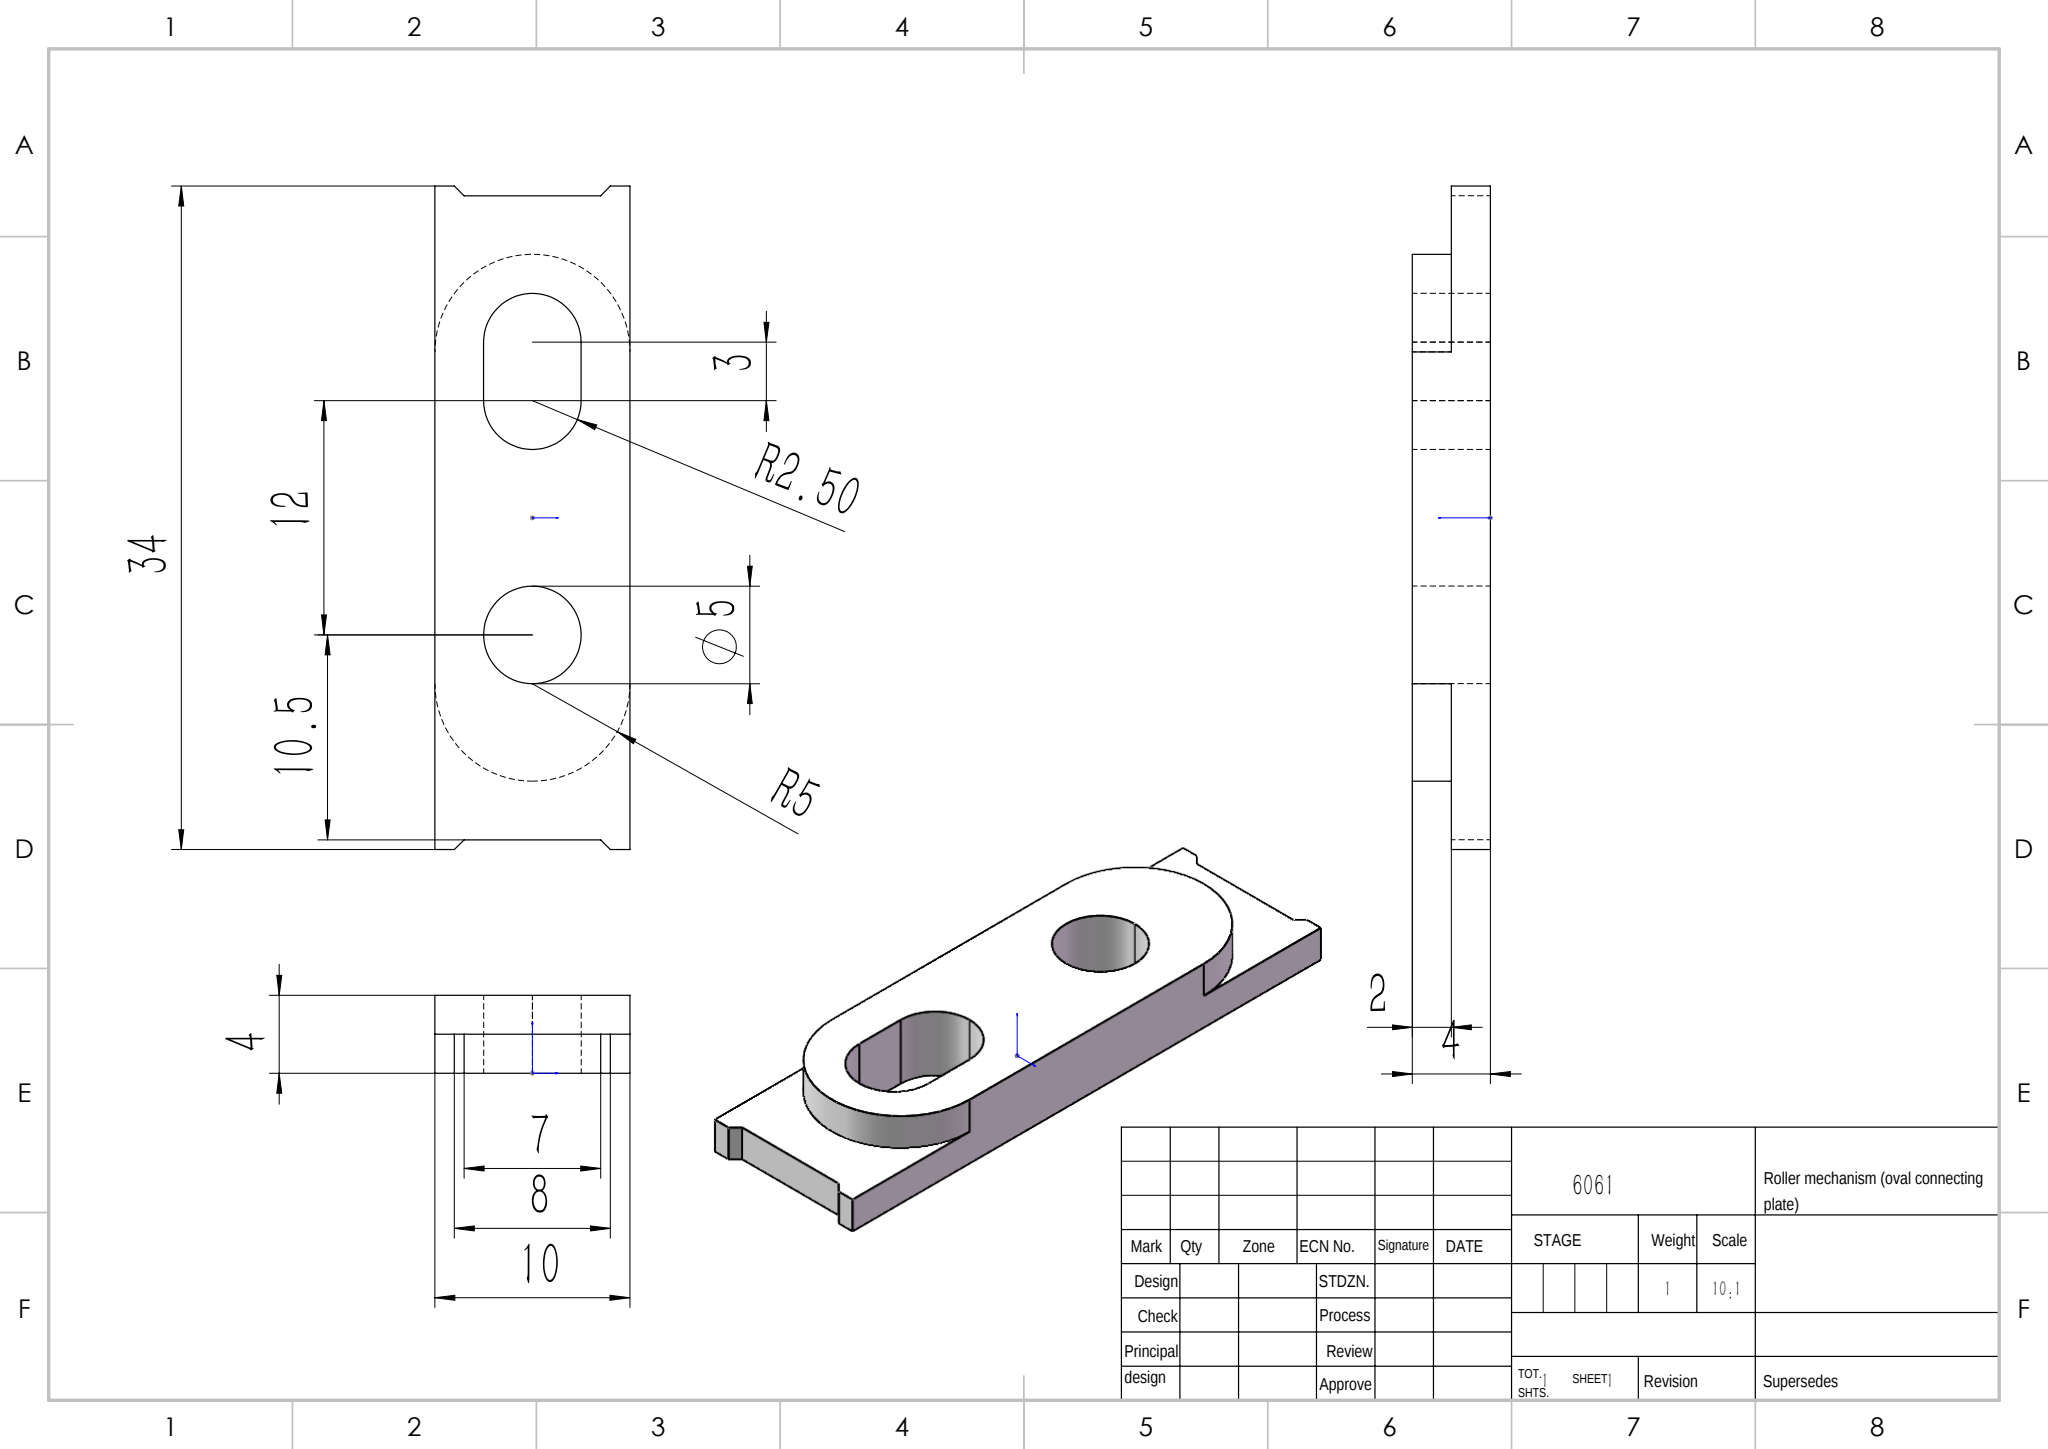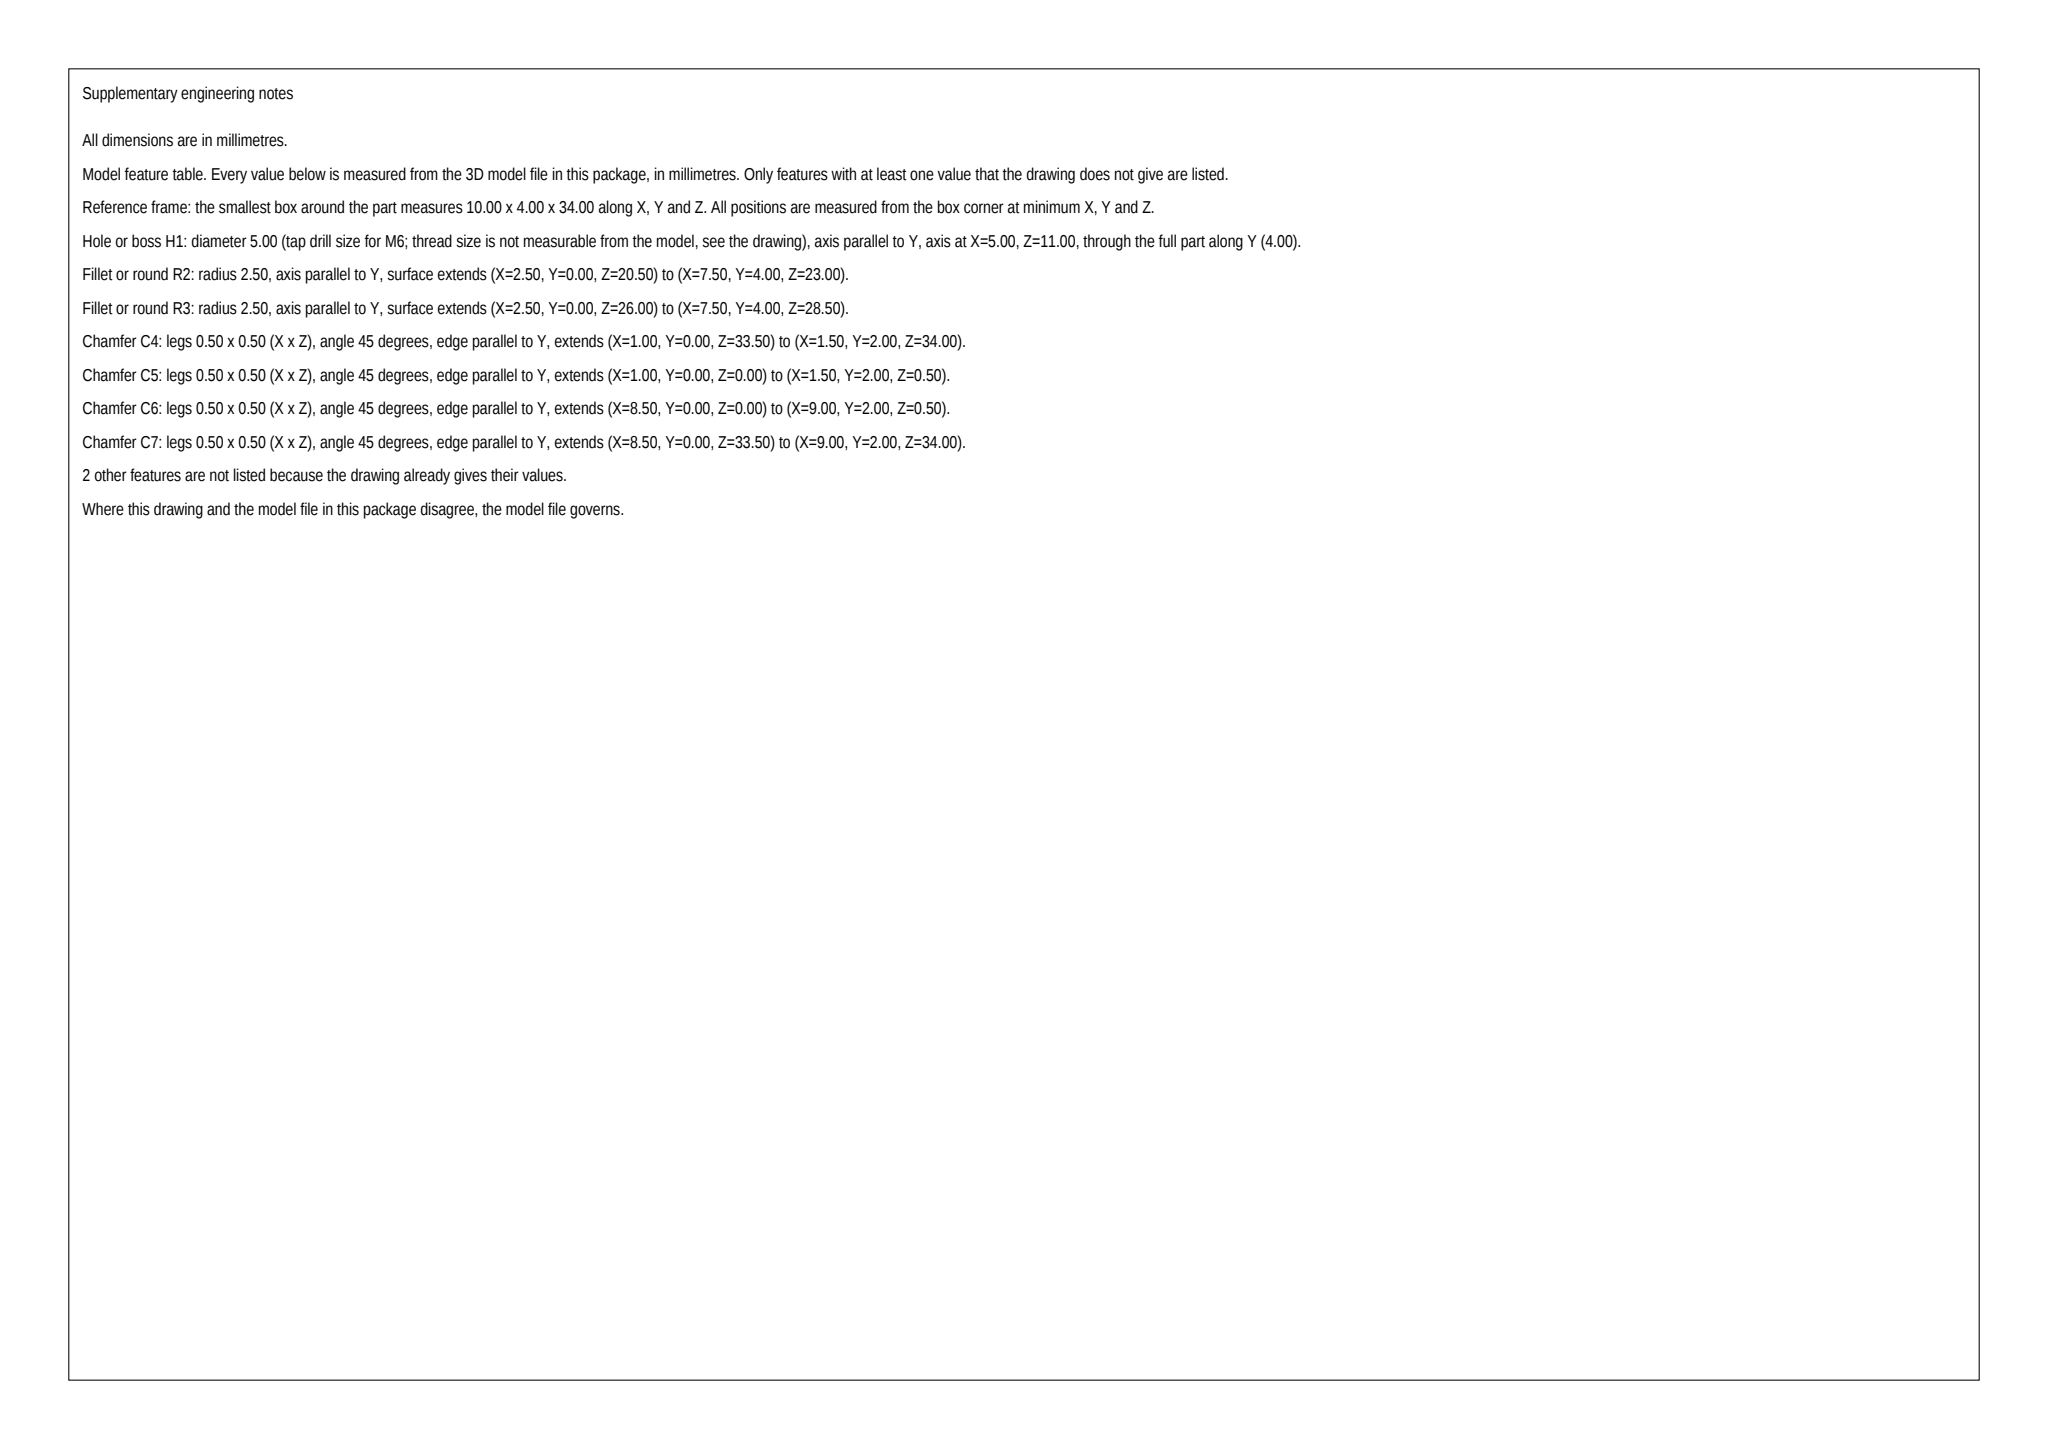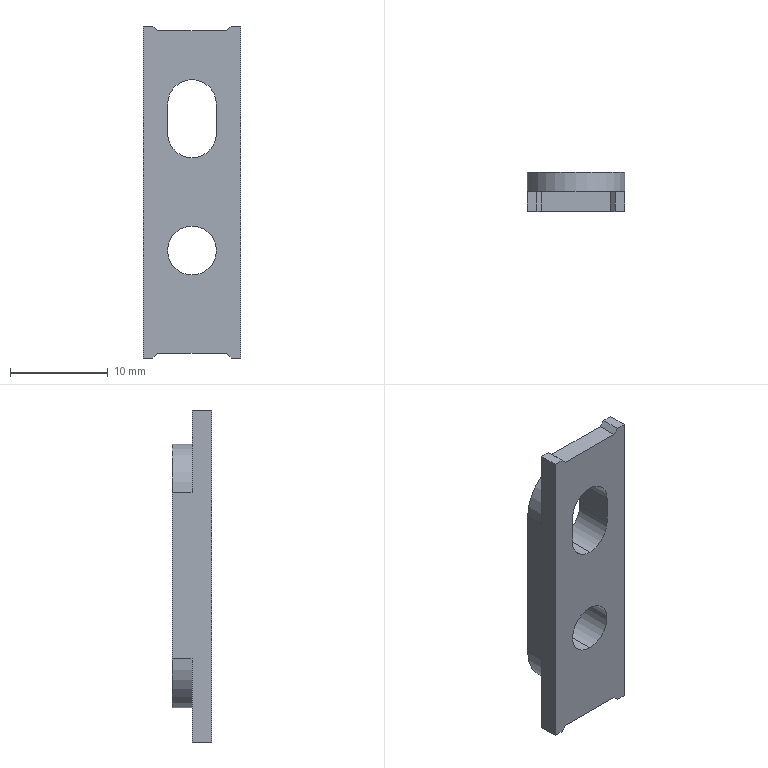Part | SolidWorks | mm | material 6061 | 1 solid | 26 faces | box 10 x 4 x 34 mm | volume 945 mm3 | plane 18 | cylinder 8 | commonest cylinder face diameters 5 x5 10 x3
STEP:
#1=CARTESIAN_POINT('',(2.5,4.,6.));
#2=VERTEX_POINT('',#1);
#3=CARTESIAN_POINT('',(2.5,0.,6.));
#4=VERTEX_POINT('',#3);
#5=CARTESIAN_POINT('',(2.5,4.,6.));
#6=DIRECTION('',(0.,-1.,0.));
#7=VECTOR('',#6,1000.);
#8=LINE('',#5,#7);
#9=EDGE_CURVE('',#2,#4,#8,.T.);
#10=ORIENTED_EDGE('',*,*,#9,.T.);
#11=CARTESIAN_POINT('',(2.5,0.,9.));
#12=VERTEX_POINT('',#11);
#13=CARTESIAN_POINT('',(2.5,0.,-0.));
#14=DIRECTION('',(0.,0.,1.));
#15=VECTOR('',#14,1000.);
#16=LINE('',#13,#15);
#17=EDGE_CURVE('',#4,#12,#16,.T.);
#18=ORIENTED_EDGE('',*,*,#17,.T.);
#19=CARTESIAN_POINT('',(2.5,4.,9.));
#20=VERTEX_POINT('',#19);
#21=CARTESIAN_POINT('',(2.5,4.,9.));
#22=DIRECTION('',(0.,-1.,0.));
#23=VECTOR('',#22,1000.);
#24=LINE('',#21,#23);
#25=EDGE_CURVE('',#20,#12,#24,.T.);
#26=ORIENTED_EDGE('',*,*,#25,.F.);
#27=CARTESIAN_POINT('',(2.5,4.,6.));
#28=DIRECTION('',(-0.,0.,-1.));
#29=VECTOR('',#28,1000.);
#30=LINE('',#27,#29);
#31=EDGE_CURVE('',#20,#2,#30,.T.);
#32=ORIENTED_EDGE('',*,*,#31,.T.);
#33=EDGE_LOOP('',(#10,#18,#26,#32));
#34=FACE_OUTER_BOUND('',#33,.T.);
#35=CARTESIAN_POINT('',(2.5,4.,6.));
#36=DIRECTION('',(-1.,0.,0.));
#37=DIRECTION('',(0.,1.,0.));
#38=AXIS2_PLACEMENT_3D('',#35,#36,#37);
#39=PLANE('',#38);
#40=ADVANCED_FACE('',(#34),#39,.T.);
#41=ORIENTED_EDGE('',*,*,#25,.T.);
#42=CARTESIAN_POINT('',(-2.5,0.,9.));
#43=VERTEX_POINT('',#42);
#44=CARTESIAN_POINT('',(0.,0.,9.));
#45=DIRECTION('',(0.,1.,0.));
#46=DIRECTION('',(0.,0.,1.));
#47=AXIS2_PLACEMENT_3D('',#44,#45,#46);
#48=CIRCLE('',#47,2.5);
#49=EDGE_CURVE('',#43,#12,#48,.T.);
#50=ORIENTED_EDGE('',*,*,#49,.F.);
#51=CARTESIAN_POINT('',(-2.5,4.,9.));
#52=VERTEX_POINT('',#51);
#53=CARTESIAN_POINT('',(-2.5,4.,9.));
#54=DIRECTION('',(0.,-1.,0.));
#55=VECTOR('',#54,1000.);
#56=LINE('',#53,#55);
#57=EDGE_CURVE('',#52,#43,#56,.T.);
#58=ORIENTED_EDGE('',*,*,#57,.F.);
#59=CARTESIAN_POINT('',(0.,4.,9.));
#60=DIRECTION('',(0.,1.,0.));
#61=DIRECTION('',(0.,0.,1.));
#62=AXIS2_PLACEMENT_3D('',#59,#60,#61);
#63=CIRCLE('',#62,2.5);
#64=EDGE_CURVE('',#52,#20,#63,.T.);
#65=ORIENTED_EDGE('',*,*,#64,.T.);
#66=EDGE_LOOP('',(#41,#50,#58,#65));
#67=FACE_OUTER_BOUND('',#66,.T.);
#68=CARTESIAN_POINT('',(0.,4.,9.));
#69=DIRECTION('',(0.,-1.,0.));
#70=DIRECTION('',(0.,0.,-1.));
#71=AXIS2_PLACEMENT_3D('',#68,#69,#70);
#72=CYLINDRICAL_SURFACE('',#71,2.5);
#73=ADVANCED_FACE('',(#67),#72,.F.);
#74=ORIENTED_EDGE('',*,*,#57,.T.);
#75=CARTESIAN_POINT('',(-2.5,0.,6.));
#76=VERTEX_POINT('',#75);
#77=CARTESIAN_POINT('',(-2.5,0.,0.));
#78=DIRECTION('',(0.,0.,1.));
#79=VECTOR('',#78,1000.);
#80=LINE('',#77,#79);
#81=EDGE_CURVE('',#76,#43,#80,.T.);
#82=ORIENTED_EDGE('',*,*,#81,.F.);
#83=CARTESIAN_POINT('',(-2.5,4.,6.));
#84=VERTEX_POINT('',#83);
#85=CARTESIAN_POINT('',(-2.5,4.,6.));
#86=DIRECTION('',(0.,-1.,0.));
#87=VECTOR('',#86,1000.);
#88=LINE('',#85,#87);
#89=EDGE_CURVE('',#84,#76,#88,.T.);
#90=ORIENTED_EDGE('',*,*,#89,.F.);
#91=CARTESIAN_POINT('',(-2.5,4.,6.));
#92=DIRECTION('',(0.,0.,1.));
#93=VECTOR('',#92,1000.);
#94=LINE('',#91,#93);
#95=EDGE_CURVE('',#84,#52,#94,.T.);
#96=ORIENTED_EDGE('',*,*,#95,.T.);
#97=EDGE_LOOP('',(#74,#82,#90,#96));
#98=FACE_OUTER_BOUND('',#97,.T.);
#99=CARTESIAN_POINT('',(-2.5,4.,6.));
#100=DIRECTION('',(1.,0.,-0.));
#101=DIRECTION('',(-0.,0.,-1.));
#102=AXIS2_PLACEMENT_3D('',#99,#100,#101);
#103=PLANE('',#102);
#104=ADVANCED_FACE('',(#98),#103,.T.);
#105=CARTESIAN_POINT('',(0.,4.,3.5));
#106=VERTEX_POINT('',#105);
#107=CARTESIAN_POINT('',(0.,0.,3.5));
#108=VERTEX_POINT('',#107);
#109=CARTESIAN_POINT('',(0.,4.,3.5));
#110=DIRECTION('',(0.,-1.,0.));
#111=VECTOR('',#110,1000.);
#112=LINE('',#109,#111);
#113=EDGE_CURVE('',#106,#108,#112,.T.);
#114=ORIENTED_EDGE('',*,*,#113,.F.);
#115=CARTESIAN_POINT('',(0.,4.,6.));
#116=DIRECTION('',(0.,1.,0.));
#117=DIRECTION('',(0.,0.,1.));
#118=AXIS2_PLACEMENT_3D('',#115,#116,#117);
#119=CIRCLE('',#118,2.5);
#120=EDGE_CURVE('',#106,#84,#119,.T.);
#121=ORIENTED_EDGE('',*,*,#120,.T.);
#122=ORIENTED_EDGE('',*,*,#89,.T.);
#123=CARTESIAN_POINT('',(0.,0.,6.));
#124=DIRECTION('',(0.,1.,0.));
#125=DIRECTION('',(0.,0.,1.));
#126=AXIS2_PLACEMENT_3D('',#123,#124,#125);
#127=CIRCLE('',#126,2.5);
#128=EDGE_CURVE('',#108,#76,#127,.T.);
#129=ORIENTED_EDGE('',*,*,#128,.F.);
#130=EDGE_LOOP('',(#114,#121,#122,#129));
#131=FACE_OUTER_BOUND('',#130,.T.);
#132=CARTESIAN_POINT('',(0.,4.,6.));
#133=DIRECTION('',(0.,-1.,0.));
#134=DIRECTION('',(0.,0.,-1.));
#135=AXIS2_PLACEMENT_3D('',#132,#133,#134);
#136=CYLINDRICAL_SURFACE('',#135,2.5);
#137=ADVANCED_FACE('',(#131),#136,.F.);
#138=CARTESIAN_POINT('',(0.,4.,-3.5));
#139=VERTEX_POINT('',#138);
#140=CARTESIAN_POINT('',(0.,0.,-3.5));
#141=VERTEX_POINT('',#140);
#142=CARTESIAN_POINT('',(0.,4.,-3.5));
#143=DIRECTION('',(0.,-1.,0.));
#144=VECTOR('',#143,1000.);
#145=LINE('',#142,#144);
#146=EDGE_CURVE('',#139,#141,#145,.T.);
#147=ORIENTED_EDGE('',*,*,#146,.F.);
#148=CARTESIAN_POINT('',(0.,4.,-8.5));
#149=VERTEX_POINT('',#148);
#150=CARTESIAN_POINT('',(0.,4.,-6.));
#151=DIRECTION('',(0.,1.,0.));
#152=DIRECTION('',(0.,0.,1.));
#153=AXIS2_PLACEMENT_3D('',#150,#151,#152);
#154=CIRCLE('',#153,2.5);
#155=EDGE_CURVE('',#139,#149,#154,.T.);
#156=ORIENTED_EDGE('',*,*,#155,.T.);
#157=CARTESIAN_POINT('',(0.,0.,-8.5));
#158=VERTEX_POINT('',#157);
#159=CARTESIAN_POINT('',(0.,4.,-8.5));
#160=DIRECTION('',(0.,-1.,0.));
#161=VECTOR('',#160,1000.);
#162=LINE('',#159,#161);
#163=EDGE_CURVE('',#149,#158,#162,.T.);
#164=ORIENTED_EDGE('',*,*,#163,.T.);
#165=CARTESIAN_POINT('',(0.,0.,-6.));
#166=DIRECTION('',(0.,1.,0.));
#167=DIRECTION('',(0.,0.,1.));
#168=AXIS2_PLACEMENT_3D('',#165,#166,#167);
#169=CIRCLE('',#168,2.5);
#170=EDGE_CURVE('',#141,#158,#169,.T.);
#171=ORIENTED_EDGE('',*,*,#170,.F.);
#172=EDGE_LOOP('',(#147,#156,#164,#171));
#173=FACE_OUTER_BOUND('',#172,.T.);
#174=CARTESIAN_POINT('',(0.,4.,-6.));
#175=DIRECTION('',(0.,-1.,0.));
#176=DIRECTION('',(0.,0.,-1.));
#177=AXIS2_PLACEMENT_3D('',#174,#175,#176);
#178=CYLINDRICAL_SURFACE('',#177,2.5);
#179=ADVANCED_FACE('',(#173),#178,.F.);
#180=CARTESIAN_POINT('',(-5.,2.,8.5));
#181=VERTEX_POINT('',#180);
#182=CARTESIAN_POINT('',(5.,2.,8.5));
#183=VERTEX_POINT('',#182);
#184=CARTESIAN_POINT('',(0.,2.,8.5));
#185=DIRECTION('',(0.,1.,0.));
#186=DIRECTION('',(0.,0.,1.));
#187=AXIS2_PLACEMENT_3D('',#184,#185,#186);
#188=CIRCLE('',#187,5.);
#189=EDGE_CURVE('',#181,#183,#188,.T.);
#190=ORIENTED_EDGE('',*,*,#189,.T.);
#191=CARTESIAN_POINT('',(5.,4.,8.5));
#192=VERTEX_POINT('',#191);
#193=CARTESIAN_POINT('',(5.,4.,8.5));
#194=DIRECTION('',(0.,-1.,0.));
#195=VECTOR('',#194,1000.);
#196=LINE('',#193,#195);
#197=EDGE_CURVE('',#192,#183,#196,.T.);
#198=ORIENTED_EDGE('',*,*,#197,.F.);
#199=CARTESIAN_POINT('',(-5.,4.,8.5));
#200=VERTEX_POINT('',#199);
#201=CARTESIAN_POINT('',(0.,4.,8.5));
#202=DIRECTION('',(0.,1.,0.));
#203=DIRECTION('',(0.,0.,1.));
#204=AXIS2_PLACEMENT_3D('',#201,#202,#203);
#205=CIRCLE('',#204,5.);
#206=EDGE_CURVE('',#200,#192,#205,.T.);
#207=ORIENTED_EDGE('',*,*,#206,.F.);
#208=CARTESIAN_POINT('',(-5.,4.,8.5));
#209=DIRECTION('',(0.,-1.,0.));
#210=VECTOR('',#209,1000.);
#211=LINE('',#208,#210);
#212=EDGE_CURVE('',#200,#181,#211,.T.);
#213=ORIENTED_EDGE('',*,*,#212,.T.);
#214=EDGE_LOOP('',(#190,#198,#207,#213));
#215=FACE_OUTER_BOUND('',#214,.T.);
#216=CARTESIAN_POINT('',(0.,4.,8.5));
#217=DIRECTION('',(0.,-1.,0.));
#218=DIRECTION('',(0.,0.,-1.));
#219=AXIS2_PLACEMENT_3D('',#216,#217,#218);
#220=CYLINDRICAL_SURFACE('',#219,5.);
#221=ADVANCED_FACE('',(#215),#220,.T.);
#222=CARTESIAN_POINT('',(0.,4.,-13.5));
#223=VERTEX_POINT('',#222);
#224=CARTESIAN_POINT('',(0.,2.,-13.5));
#225=VERTEX_POINT('',#224);
#226=CARTESIAN_POINT('',(0.,4.,-13.5));
#227=DIRECTION('',(0.,-1.,0.));
#228=VECTOR('',#227,1000.);
#229=LINE('',#226,#228);
#230=EDGE_CURVE('',#223,#225,#229,.T.);
#231=ORIENTED_EDGE('',*,*,#230,.F.);
#232=CARTESIAN_POINT('',(5.,4.,-8.5));
#233=VERTEX_POINT('',#232);
#234=CARTESIAN_POINT('',(0.,4.,-8.5));
#235=DIRECTION('',(0.,1.,0.));
#236=DIRECTION('',(0.,0.,1.));
#237=AXIS2_PLACEMENT_3D('',#234,#235,#236);
#238=CIRCLE('',#237,5.);
#239=EDGE_CURVE('',#233,#223,#238,.T.);
#240=ORIENTED_EDGE('',*,*,#239,.F.);
#241=CARTESIAN_POINT('',(5.,2.,-8.5));
#242=VERTEX_POINT('',#241);
#243=CARTESIAN_POINT('',(5.,4.,-8.5));
#244=DIRECTION('',(0.,-1.,0.));
#245=VECTOR('',#244,1000.);
#246=LINE('',#243,#245);
#247=EDGE_CURVE('',#233,#242,#246,.T.);
#248=ORIENTED_EDGE('',*,*,#247,.T.);
#249=CARTESIAN_POINT('',(0.,2.,-8.5));
#250=DIRECTION('',(0.,1.,0.));
#251=DIRECTION('',(0.,0.,1.));
#252=AXIS2_PLACEMENT_3D('',#249,#250,#251);
#253=CIRCLE('',#252,5.);
#254=EDGE_CURVE('',#242,#225,#253,.T.);
#255=ORIENTED_EDGE('',*,*,#254,.T.);
#256=EDGE_LOOP('',(#231,#240,#248,#255));
#257=FACE_OUTER_BOUND('',#256,.T.);
#258=CARTESIAN_POINT('',(0.,4.,-8.5));
#259=DIRECTION('',(0.,-1.,0.));
#260=DIRECTION('',(0.,0.,-1.));
#261=AXIS2_PLACEMENT_3D('',#258,#259,#260);
#262=CYLINDRICAL_SURFACE('',#261,5.);
#263=ADVANCED_FACE('',(#257),#262,.T.);
#264=ORIENTED_EDGE('',*,*,#95,.F.);
#265=ORIENTED_EDGE('',*,*,#120,.F.);
#266=CARTESIAN_POINT('',(0.,4.,6.));
#267=DIRECTION('',(0.,1.,0.));
#268=DIRECTION('',(0.,0.,1.));
#269=AXIS2_PLACEMENT_3D('',#266,#267,#268);
#270=CIRCLE('',#269,2.5);
#271=EDGE_CURVE('',#2,#106,#270,.T.);
#272=ORIENTED_EDGE('',*,*,#271,.F.);
#273=ORIENTED_EDGE('',*,*,#31,.F.);
#274=ORIENTED_EDGE('',*,*,#64,.F.);
#275=EDGE_LOOP('',(#264,#265,#272,#273,#274));
#276=FACE_BOUND('',#275,.T.);
#277=CARTESIAN_POINT('',(0.,4.,-6.));
#278=DIRECTION('',(0.,1.,0.));
#279=DIRECTION('',(0.,0.,1.));
#280=AXIS2_PLACEMENT_3D('',#277,#278,#279);
#281=CIRCLE('',#280,2.5);
#282=EDGE_CURVE('',#149,#139,#281,.T.);
#283=ORIENTED_EDGE('',*,*,#282,.F.);
#284=ORIENTED_EDGE('',*,*,#155,.F.);
#285=EDGE_LOOP('',(#283,#284));
#286=FACE_BOUND('',#285,.T.);
#287=ORIENTED_EDGE('',*,*,#239,.T.);
#288=CARTESIAN_POINT('',(-5.,4.,-8.5));
#289=VERTEX_POINT('',#288);
#290=CARTESIAN_POINT('',(0.,4.,-8.5));
#291=DIRECTION('',(0.,1.,0.));
#292=DIRECTION('',(0.,0.,1.));
#293=AXIS2_PLACEMENT_3D('',#290,#291,#292);
#294=CIRCLE('',#293,5.);
#295=EDGE_CURVE('',#223,#289,#294,.T.);
#296=ORIENTED_EDGE('',*,*,#295,.T.);
#297=CARTESIAN_POINT('',(-5.,4.,-8.5));
#298=DIRECTION('',(0.,0.,1.));
#299=VECTOR('',#298,1000.);
#300=LINE('',#297,#299);
#301=EDGE_CURVE('',#289,#200,#300,.T.);
#302=ORIENTED_EDGE('',*,*,#301,.T.);
#303=ORIENTED_EDGE('',*,*,#206,.T.);
#304=CARTESIAN_POINT('',(5.,4.,-8.5));
#305=DIRECTION('',(-0.,0.,-1.));
#306=VECTOR('',#305,1000.);
#307=LINE('',#304,#306);
#308=EDGE_CURVE('',#192,#233,#307,.T.);
#309=ORIENTED_EDGE('',*,*,#308,.T.);
#310=EDGE_LOOP('',(#287,#296,#302,#303,#309));
#311=FACE_OUTER_BOUND('',#310,.T.);
#312=CARTESIAN_POINT('',(0.,4.,-8.5));
#313=DIRECTION('',(0.,1.,0.));
#314=DIRECTION('',(1.,0.,0.));
#315=AXIS2_PLACEMENT_3D('',#312,#313,#314);
#316=PLANE('',#315);
#317=ADVANCED_FACE('',(#276,#286,#311),#316,.T.);
#318=CARTESIAN_POINT('',(0.,0.,-6.));
#319=DIRECTION('',(0.,1.,0.));
#320=DIRECTION('',(0.,0.,1.));
#321=AXIS2_PLACEMENT_3D('',#318,#319,#320);
#322=CIRCLE('',#321,2.5);
#323=EDGE_CURVE('',#158,#141,#322,.T.);
#324=ORIENTED_EDGE('',*,*,#323,.T.);
#325=ORIENTED_EDGE('',*,*,#170,.T.);
#326=EDGE_LOOP('',(#324,#325));
#327=FACE_BOUND('',#326,.T.);
#328=ORIENTED_EDGE('',*,*,#81,.T.);
#329=ORIENTED_EDGE('',*,*,#49,.T.);
#330=ORIENTED_EDGE('',*,*,#17,.F.);
#331=CARTESIAN_POINT('',(0.,0.,6.));
#332=DIRECTION('',(0.,1.,0.));
#333=DIRECTION('',(0.,0.,1.));
#334=AXIS2_PLACEMENT_3D('',#331,#332,#333);
#335=CIRCLE('',#334,2.5);
#336=EDGE_CURVE('',#4,#108,#335,.T.);
#337=ORIENTED_EDGE('',*,*,#336,.T.);
#338=ORIENTED_EDGE('',*,*,#128,.T.);
#339=EDGE_LOOP('',(#328,#329,#330,#337,#338));
#340=FACE_BOUND('',#339,.T.);
#341=CARTESIAN_POINT('',(-3.5,0.,16.5));
#342=VERTEX_POINT('',#341);
#343=CARTESIAN_POINT('',(3.5,0.,16.5));
#344=VERTEX_POINT('',#343);
#345=CARTESIAN_POINT('',(-3.5,0.,16.5));
#346=DIRECTION('',(1.,0.,0.));
#347=VECTOR('',#346,1000.);
#348=LINE('',#345,#347);
#349=EDGE_CURVE('',#342,#344,#348,.T.);
#350=ORIENTED_EDGE('',*,*,#349,.F.);
#351=CARTESIAN_POINT('',(-4.,0.,17.));
#352=VERTEX_POINT('',#351);
#353=CARTESIAN_POINT('',(-3.5,0.,16.5));
#354=DIRECTION('',(0.7071,0.,-0.7071));
#355=VECTOR('',#354,1000.);
#356=LINE('',#353,#355);
#357=EDGE_CURVE('',#352,#342,#356,.T.);
#358=ORIENTED_EDGE('',*,*,#357,.F.);
#359=CARTESIAN_POINT('',(-5.,0.,17.));
#360=VERTEX_POINT('',#359);
#361=CARTESIAN_POINT('',(-4.,0.,17.));
#362=DIRECTION('',(1.,0.,0.));
#363=VECTOR('',#362,1000.);
#364=LINE('',#361,#363);
#365=EDGE_CURVE('',#360,#352,#364,.T.);
#366=ORIENTED_EDGE('',*,*,#365,.F.);
#367=CARTESIAN_POINT('',(-5.,0.,-17.));
#368=VERTEX_POINT('',#367);
#369=CARTESIAN_POINT('',(-5.,0.,-17.));
#370=DIRECTION('',(0.,0.,1.));
#371=VECTOR('',#370,1000.);
#372=LINE('',#369,#371);
#373=EDGE_CURVE('',#368,#360,#372,.T.);
#374=ORIENTED_EDGE('',*,*,#373,.F.);
#375=CARTESIAN_POINT('',(-4.,0.,-17.));
#376=VERTEX_POINT('',#375);
#377=CARTESIAN_POINT('',(-4.,0.,-17.));
#378=DIRECTION('',(-1.,0.,0.));
#379=VECTOR('',#378,1000.);
#380=LINE('',#377,#379);
#381=EDGE_CURVE('',#376,#368,#380,.T.);
#382=ORIENTED_EDGE('',*,*,#381,.F.);
#383=CARTESIAN_POINT('',(-3.5,0.,-16.5));
#384=VERTEX_POINT('',#383);
#385=CARTESIAN_POINT('',(-3.5,0.,-16.5));
#386=DIRECTION('',(-0.7071,0.,-0.7071));
#387=VECTOR('',#386,1000.);
#388=LINE('',#385,#387);
#389=EDGE_CURVE('',#384,#376,#388,.T.);
#390=ORIENTED_EDGE('',*,*,#389,.F.);
#391=CARTESIAN_POINT('',(3.5,0.,-16.5));
#392=VERTEX_POINT('',#391);
#393=CARTESIAN_POINT('',(-3.5,0.,-16.5));
#394=DIRECTION('',(-1.,0.,0.));
#395=VECTOR('',#394,1000.);
#396=LINE('',#393,#395);
#397=EDGE_CURVE('',#392,#384,#396,.T.);
#398=ORIENTED_EDGE('',*,*,#397,.F.);
#399=CARTESIAN_POINT('',(4.,0.,-17.));
#400=VERTEX_POINT('',#399);
#401=CARTESIAN_POINT('',(3.5,0.,-16.5));
#402=DIRECTION('',(-0.7071,0.,0.7071));
#403=VECTOR('',#402,1000.);
#404=LINE('',#401,#403);
#405=EDGE_CURVE('',#400,#392,#404,.T.);
#406=ORIENTED_EDGE('',*,*,#405,.F.);
#407=CARTESIAN_POINT('',(5.,0.,-17.));
#408=VERTEX_POINT('',#407);
#409=CARTESIAN_POINT('',(4.,0.,-17.));
#410=DIRECTION('',(-1.,0.,0.));
#411=VECTOR('',#410,1000.);
#412=LINE('',#409,#411);
#413=EDGE_CURVE('',#408,#400,#412,.T.);
#414=ORIENTED_EDGE('',*,*,#413,.F.);
#415=CARTESIAN_POINT('',(5.,0.,17.));
#416=VERTEX_POINT('',#415);
#417=CARTESIAN_POINT('',(5.,0.,-17.));
#418=DIRECTION('',(0.,0.,-1.));
#419=VECTOR('',#418,1000.);
#420=LINE('',#417,#419);
#421=EDGE_CURVE('',#416,#408,#420,.T.);
#422=ORIENTED_EDGE('',*,*,#421,.F.);
#423=CARTESIAN_POINT('',(4.,0.,17.));
#424=VERTEX_POINT('',#423);
#425=CARTESIAN_POINT('',(4.,0.,17.));
#426=DIRECTION('',(1.,0.,0.));
#427=VECTOR('',#426,1000.);
#428=LINE('',#425,#427);
#429=EDGE_CURVE('',#424,#416,#428,.T.);
#430=ORIENTED_EDGE('',*,*,#429,.F.);
#431=CARTESIAN_POINT('',(3.5,0.,16.5));
#432=DIRECTION('',(0.7071,0.,0.7071));
#433=VECTOR('',#432,1000.);
#434=LINE('',#431,#433);
#435=EDGE_CURVE('',#344,#424,#434,.T.);
#436=ORIENTED_EDGE('',*,*,#435,.F.);
#437=EDGE_LOOP('',(#350,#358,#366,#374,#382,#390,#398,#406,#414,#422,#430,#436));
#438=FACE_OUTER_BOUND('',#437,.T.);
#439=CARTESIAN_POINT('',(0.,0.,0.));
#440=DIRECTION('',(0.,-1.,0.));
#441=DIRECTION('',(0.,0.,-1.));
#442=AXIS2_PLACEMENT_3D('',#439,#440,#441);
#443=PLANE('',#442);
#444=ADVANCED_FACE('',(#327,#340,#438),#443,.T.);
#445=ORIENTED_EDGE('',*,*,#357,.T.);
#446=CARTESIAN_POINT('',(-3.5,2.,16.5));
#447=VERTEX_POINT('',#446);
#448=CARTESIAN_POINT('',(-3.5,2.,16.5));
#449=DIRECTION('',(0.,-1.,0.));
#450=VECTOR('',#449,1000.);
#451=LINE('',#448,#450);
#452=EDGE_CURVE('',#447,#342,#451,.T.);
#453=ORIENTED_EDGE('',*,*,#452,.F.);
#454=CARTESIAN_POINT('',(-4.,2.,17.));
#455=VERTEX_POINT('',#454);
#456=CARTESIAN_POINT('',(-3.5,2.,16.5));
#457=DIRECTION('',(0.7071,0.,-0.7071));
#458=VECTOR('',#457,1000.);
#459=LINE('',#456,#458);
#460=EDGE_CURVE('',#455,#447,#459,.T.);
#461=ORIENTED_EDGE('',*,*,#460,.F.);
#462=CARTESIAN_POINT('',(-4.,2.,17.));
#463=DIRECTION('',(0.,-1.,0.));
#464=VECTOR('',#463,1000.);
#465=LINE('',#462,#464);
#466=EDGE_CURVE('',#455,#352,#465,.T.);
#467=ORIENTED_EDGE('',*,*,#466,.T.);
#468=EDGE_LOOP('',(#445,#453,#461,#467));
#469=FACE_OUTER_BOUND('',#468,.T.);
#470=CARTESIAN_POINT('',(-3.5,2.,16.5));
#471=DIRECTION('',(-0.7071,0.,-0.7071));
#472=DIRECTION('',(-0.7071,0.,0.7071));
#473=AXIS2_PLACEMENT_3D('',#470,#471,#472);
#474=PLANE('',#473);
#475=ADVANCED_FACE('',(#469),#474,.F.);
#476=ORIENTED_EDGE('',*,*,#365,.T.);
#477=ORIENTED_EDGE('',*,*,#466,.F.);
#478=CARTESIAN_POINT('',(-5.,2.,17.));
#479=VERTEX_POINT('',#478);
#480=CARTESIAN_POINT('',(-4.,2.,17.));
#481=DIRECTION('',(1.,0.,0.));
#482=VECTOR('',#481,1000.);
#483=LINE('',#480,#482);
#484=EDGE_CURVE('',#479,#455,#483,.T.);
#485=ORIENTED_EDGE('',*,*,#484,.F.);
#486=CARTESIAN_POINT('',(-5.,2.,17.));
#487=DIRECTION('',(0.,-1.,0.));
#488=VECTOR('',#487,1000.);
#489=LINE('',#486,#488);
#490=EDGE_CURVE('',#479,#360,#489,.T.);
#491=ORIENTED_EDGE('',*,*,#490,.T.);
#492=EDGE_LOOP('',(#476,#477,#485,#491));
#493=FACE_OUTER_BOUND('',#492,.T.);
#494=CARTESIAN_POINT('',(-4.,2.,17.));
#495=DIRECTION('',(0.,0.,-1.));
#496=DIRECTION('',(0.,-1.,0.));
#497=AXIS2_PLACEMENT_3D('',#494,#495,#496);
#498=PLANE('',#497);
#499=ADVANCED_FACE('',(#493),#498,.F.);
#500=ORIENTED_EDGE('',*,*,#373,.T.);
#501=ORIENTED_EDGE('',*,*,#490,.F.);
#502=CARTESIAN_POINT('',(-5.,2.,-17.));
#503=DIRECTION('',(0.,0.,1.));
#504=VECTOR('',#503,1000.);
#505=LINE('',#502,#504);
#506=EDGE_CURVE('',#181,#479,#505,.T.);
#507=ORIENTED_EDGE('',*,*,#506,.F.);
#508=ORIENTED_EDGE('',*,*,#212,.F.);
#509=ORIENTED_EDGE('',*,*,#301,.F.);
#510=CARTESIAN_POINT('',(-5.,2.,-8.5));
#511=VERTEX_POINT('',#510);
#512=CARTESIAN_POINT('',(-5.,4.,-8.5));
#513=DIRECTION('',(0.,-1.,0.));
#514=VECTOR('',#513,1000.);
#515=LINE('',#512,#514);
#516=EDGE_CURVE('',#289,#511,#515,.T.);
#517=ORIENTED_EDGE('',*,*,#516,.T.);
#518=CARTESIAN_POINT('',(-5.,2.,-17.));
#519=VERTEX_POINT('',#518);
#520=CARTESIAN_POINT('',(-5.,2.,-17.));
#521=DIRECTION('',(0.,0.,1.));
#522=VECTOR('',#521,1000.);
#523=LINE('',#520,#522);
#524=EDGE_CURVE('',#519,#511,#523,.T.);
#525=ORIENTED_EDGE('',*,*,#524,.F.);
#526=CARTESIAN_POINT('',(-5.,2.,-17.));
#527=DIRECTION('',(0.,-1.,0.));
#528=VECTOR('',#527,1000.);
#529=LINE('',#526,#528);
#530=EDGE_CURVE('',#519,#368,#529,.T.);
#531=ORIENTED_EDGE('',*,*,#530,.T.);
#532=EDGE_LOOP('',(#500,#501,#507,#508,#509,#517,#525,#531));
#533=FACE_OUTER_BOUND('',#532,.T.);
#534=CARTESIAN_POINT('',(-5.,2.,-17.));
#535=DIRECTION('',(1.,0.,-0.));
#536=DIRECTION('',(-0.,0.,-1.));
#537=AXIS2_PLACEMENT_3D('',#534,#535,#536);
#538=PLANE('',#537);
#539=ADVANCED_FACE('',(#533),#538,.F.);
#540=ORIENTED_EDGE('',*,*,#381,.T.);
#541=ORIENTED_EDGE('',*,*,#530,.F.);
#542=CARTESIAN_POINT('',(-4.,2.,-17.));
#543=VERTEX_POINT('',#542);
#544=CARTESIAN_POINT('',(-4.,2.,-17.));
#545=DIRECTION('',(-1.,0.,0.));
#546=VECTOR('',#545,1000.);
#547=LINE('',#544,#546);
#548=EDGE_CURVE('',#543,#519,#547,.T.);
#549=ORIENTED_EDGE('',*,*,#548,.F.);
#550=CARTESIAN_POINT('',(-4.,2.,-17.));
#551=DIRECTION('',(0.,-1.,0.));
#552=VECTOR('',#551,1000.);
#553=LINE('',#550,#552);
#554=EDGE_CURVE('',#543,#376,#553,.T.);
#555=ORIENTED_EDGE('',*,*,#554,.T.);
#556=EDGE_LOOP('',(#540,#541,#549,#555));
#557=FACE_OUTER_BOUND('',#556,.T.);
#558=CARTESIAN_POINT('',(-4.,2.,-17.));
#559=DIRECTION('',(0.,0.,1.));
#560=DIRECTION('',(1.,0.,0.));
#561=AXIS2_PLACEMENT_3D('',#558,#559,#560);
#562=PLANE('',#561);
#563=ADVANCED_FACE('',(#557),#562,.F.);
#564=ORIENTED_EDGE('',*,*,#389,.T.);
#565=ORIENTED_EDGE('',*,*,#554,.F.);
#566=CARTESIAN_POINT('',(-3.5,2.,-16.5));
#567=VERTEX_POINT('',#566);
#568=CARTESIAN_POINT('',(-3.5,2.,-16.5));
#569=DIRECTION('',(-0.7071,0.,-0.7071));
#570=VECTOR('',#569,1000.);
#571=LINE('',#568,#570);
#572=EDGE_CURVE('',#567,#543,#571,.T.);
#573=ORIENTED_EDGE('',*,*,#572,.F.);
#574=CARTESIAN_POINT('',(-3.5,2.,-16.5));
#575=DIRECTION('',(0.,-1.,0.));
#576=VECTOR('',#575,1000.);
#577=LINE('',#574,#576);
#578=EDGE_CURVE('',#567,#384,#577,.T.);
#579=ORIENTED_EDGE('',*,*,#578,.T.);
#580=EDGE_LOOP('',(#564,#565,#573,#579));
#581=FACE_OUTER_BOUND('',#580,.T.);
#582=CARTESIAN_POINT('',(-3.5,2.,-16.5));
#583=DIRECTION('',(-0.7071,0.,0.7071));
#584=DIRECTION('',(0.,1.,0.));
#585=AXIS2_PLACEMENT_3D('',#582,#583,#584);
#586=PLANE('',#585);
#587=ADVANCED_FACE('',(#581),#586,.F.);
#588=ORIENTED_EDGE('',*,*,#397,.T.);
#589=ORIENTED_EDGE('',*,*,#578,.F.);
#590=CARTESIAN_POINT('',(3.5,2.,-16.5));
#591=VERTEX_POINT('',#590);
#592=CARTESIAN_POINT('',(-3.5,2.,-16.5));
#593=DIRECTION('',(-1.,0.,0.));
#594=VECTOR('',#593,1000.);
#595=LINE('',#592,#594);
#596=EDGE_CURVE('',#591,#567,#595,.T.);
#597=ORIENTED_EDGE('',*,*,#596,.F.);
#598=CARTESIAN_POINT('',(3.5,2.,-16.5));
#599=DIRECTION('',(0.,-1.,0.));
#600=VECTOR('',#599,1000.);
#601=LINE('',#598,#600);
#602=EDGE_CURVE('',#591,#392,#601,.T.);
#603=ORIENTED_EDGE('',*,*,#602,.T.);
#604=EDGE_LOOP('',(#588,#589,#597,#603));
#605=FACE_OUTER_BOUND('',#604,.T.);
#606=CARTESIAN_POINT('',(-3.5,2.,-16.5));
#607=DIRECTION('',(0.,0.,1.));
#608=DIRECTION('',(1.,0.,0.));
#609=AXIS2_PLACEMENT_3D('',#606,#607,#608);
#610=PLANE('',#609);
#611=ADVANCED_FACE('',(#605),#610,.F.);
#612=ORIENTED_EDGE('',*,*,#405,.T.);
#613=ORIENTED_EDGE('',*,*,#602,.F.);
#614=CARTESIAN_POINT('',(4.,2.,-17.));
#615=VERTEX_POINT('',#614);
#616=CARTESIAN_POINT('',(3.5,2.,-16.5));
#617=DIRECTION('',(-0.7071,0.,0.7071));
#618=VECTOR('',#617,1000.);
#619=LINE('',#616,#618);
#620=EDGE_CURVE('',#615,#591,#619,.T.);
#621=ORIENTED_EDGE('',*,*,#620,.F.);
#622=CARTESIAN_POINT('',(4.,2.,-17.));
#623=DIRECTION('',(0.,-1.,0.));
#624=VECTOR('',#623,1000.);
#625=LINE('',#622,#624);
#626=EDGE_CURVE('',#615,#400,#625,.T.);
#627=ORIENTED_EDGE('',*,*,#626,.T.);
#628=EDGE_LOOP('',(#612,#613,#621,#627));
#629=FACE_OUTER_BOUND('',#628,.T.);
#630=CARTESIAN_POINT('',(3.5,2.,-16.5));
#631=DIRECTION('',(0.7071,0.,0.7071));
#632=DIRECTION('',(0.,-1.,0.));
#633=AXIS2_PLACEMENT_3D('',#630,#631,#632);
#634=PLANE('',#633);
#635=ADVANCED_FACE('',(#629),#634,.F.);
#636=ORIENTED_EDGE('',*,*,#413,.T.);
#637=ORIENTED_EDGE('',*,*,#626,.F.);
#638=CARTESIAN_POINT('',(5.,2.,-17.));
#639=VERTEX_POINT('',#638);
#640=CARTESIAN_POINT('',(4.,2.,-17.));
#641=DIRECTION('',(-1.,0.,0.));
#642=VECTOR('',#641,1000.);
#643=LINE('',#640,#642);
#644=EDGE_CURVE('',#639,#615,#643,.T.);
#645=ORIENTED_EDGE('',*,*,#644,.F.);
#646=CARTESIAN_POINT('',(5.,2.,-17.));
#647=DIRECTION('',(0.,-1.,0.));
#648=VECTOR('',#647,1000.);
#649=LINE('',#646,#648);
#650=EDGE_CURVE('',#639,#408,#649,.T.);
#651=ORIENTED_EDGE('',*,*,#650,.T.);
#652=EDGE_LOOP('',(#636,#637,#645,#651));
#653=FACE_OUTER_BOUND('',#652,.T.);
#654=CARTESIAN_POINT('',(4.,2.,-17.));
#655=DIRECTION('',(0.,0.,1.));
#656=DIRECTION('',(1.,0.,0.));
#657=AXIS2_PLACEMENT_3D('',#654,#655,#656);
#658=PLANE('',#657);
#659=ADVANCED_FACE('',(#653),#658,.F.);
#660=ORIENTED_EDGE('',*,*,#421,.T.);
#661=ORIENTED_EDGE('',*,*,#650,.F.);
#662=CARTESIAN_POINT('',(5.,2.,-17.));
#663=DIRECTION('',(0.,0.,-1.));
#664=VECTOR('',#663,1000.);
#665=LINE('',#662,#664);
#666=EDGE_CURVE('',#242,#639,#665,.T.);
#667=ORIENTED_EDGE('',*,*,#666,.F.);
#668=ORIENTED_EDGE('',*,*,#247,.F.);
#669=ORIENTED_EDGE('',*,*,#308,.F.);
#670=ORIENTED_EDGE('',*,*,#197,.T.);
#671=CARTESIAN_POINT('',(5.,2.,17.));
#672=VERTEX_POINT('',#671);
#673=CARTESIAN_POINT('',(5.,2.,-17.));
#674=DIRECTION('',(0.,0.,-1.));
#675=VECTOR('',#674,1000.);
#676=LINE('',#673,#675);
#677=EDGE_CURVE('',#672,#183,#676,.T.);
#678=ORIENTED_EDGE('',*,*,#677,.F.);
#679=CARTESIAN_POINT('',(5.,2.,17.));
#680=DIRECTION('',(0.,-1.,0.));
#681=VECTOR('',#680,1000.);
#682=LINE('',#679,#681);
#683=EDGE_CURVE('',#672,#416,#682,.T.);
#684=ORIENTED_EDGE('',*,*,#683,.T.);
#685=EDGE_LOOP('',(#660,#661,#667,#668,#669,#670,#678,#684));
#686=FACE_OUTER_BOUND('',#685,.T.);
#687=CARTESIAN_POINT('',(5.,2.,-17.));
#688=DIRECTION('',(-1.,0.,0.));
#689=DIRECTION('',(0.,0.,1.));
#690=AXIS2_PLACEMENT_3D('',#687,#688,#689);
#691=PLANE('',#690);
#692=ADVANCED_FACE('',(#686),#691,.F.);
#693=ORIENTED_EDGE('',*,*,#429,.T.);
#694=ORIENTED_EDGE('',*,*,#683,.F.);
#695=CARTESIAN_POINT('',(4.,2.,17.));
#696=VERTEX_POINT('',#695);
#697=CARTESIAN_POINT('',(4.,2.,17.));
#698=DIRECTION('',(1.,0.,0.));
#699=VECTOR('',#698,1000.);
#700=LINE('',#697,#699);
#701=EDGE_CURVE('',#696,#672,#700,.T.);
#702=ORIENTED_EDGE('',*,*,#701,.F.);
#703=CARTESIAN_POINT('',(4.,2.,17.));
#704=DIRECTION('',(0.,-1.,0.));
#705=VECTOR('',#704,1000.);
#706=LINE('',#703,#705);
#707=EDGE_CURVE('',#696,#424,#706,.T.);
#708=ORIENTED_EDGE('',*,*,#707,.T.);
#709=EDGE_LOOP('',(#693,#694,#702,#708));
#710=FACE_OUTER_BOUND('',#709,.T.);
#711=CARTESIAN_POINT('',(4.,2.,17.));
#712=DIRECTION('',(0.,0.,-1.));
#713=DIRECTION('',(0.,-1.,0.));
#714=AXIS2_PLACEMENT_3D('',#711,#712,#713);
#715=PLANE('',#714);
#716=ADVANCED_FACE('',(#710),#715,.F.);
#717=ORIENTED_EDGE('',*,*,#435,.T.);
#718=ORIENTED_EDGE('',*,*,#707,.F.);
#719=CARTESIAN_POINT('',(3.5,2.,16.5));
#720=VERTEX_POINT('',#719);
#721=CARTESIAN_POINT('',(3.5,2.,16.5));
#722=DIRECTION('',(0.7071,0.,0.7071));
#723=VECTOR('',#722,1000.);
#724=LINE('',#721,#723);
#725=EDGE_CURVE('',#720,#696,#724,.T.);
#726=ORIENTED_EDGE('',*,*,#725,.F.);
#727=CARTESIAN_POINT('',(3.5,2.,16.5));
#728=DIRECTION('',(0.,-1.,0.));
#729=VECTOR('',#728,1000.);
#730=LINE('',#727,#729);
#731=EDGE_CURVE('',#720,#344,#730,.T.);
#732=ORIENTED_EDGE('',*,*,#731,.T.);
#733=EDGE_LOOP('',(#717,#718,#726,#732));
#734=FACE_OUTER_BOUND('',#733,.T.);
#735=CARTESIAN_POINT('',(3.5,2.,16.5));
#736=DIRECTION('',(0.7071,0.,-0.7071));
#737=DIRECTION('',(0.,-1.,0.));
#738=AXIS2_PLACEMENT_3D('',#735,#736,#737);
#739=PLANE('',#738);
#740=ADVANCED_FACE('',(#734),#739,.F.);
#741=ORIENTED_EDGE('',*,*,#349,.T.);
#742=ORIENTED_EDGE('',*,*,#731,.F.);
#743=CARTESIAN_POINT('',(-3.5,2.,16.5));
#744=DIRECTION('',(1.,0.,0.));
#745=VECTOR('',#744,1000.);
#746=LINE('',#743,#745);
#747=EDGE_CURVE('',#447,#720,#746,.T.);
#748=ORIENTED_EDGE('',*,*,#747,.F.);
#749=ORIENTED_EDGE('',*,*,#452,.T.);
#750=EDGE_LOOP('',(#741,#742,#748,#749));
#751=FACE_OUTER_BOUND('',#750,.T.);
#752=CARTESIAN_POINT('',(-3.5,2.,16.5));
#753=DIRECTION('',(0.,0.,-1.));
#754=DIRECTION('',(0.,-1.,0.));
#755=AXIS2_PLACEMENT_3D('',#752,#753,#754);
#756=PLANE('',#755);
#757=ADVANCED_FACE('',(#751),#756,.F.);
#758=ORIENTED_EDGE('',*,*,#189,.F.);
#759=ORIENTED_EDGE('',*,*,#506,.T.);
#760=ORIENTED_EDGE('',*,*,#484,.T.);
#761=ORIENTED_EDGE('',*,*,#460,.T.);
#762=ORIENTED_EDGE('',*,*,#747,.T.);
#763=ORIENTED_EDGE('',*,*,#725,.T.);
#764=ORIENTED_EDGE('',*,*,#701,.T.);
#765=ORIENTED_EDGE('',*,*,#677,.T.);
#766=EDGE_LOOP('',(#758,#759,#760,#761,#762,#763,#764,#765));
#767=FACE_OUTER_BOUND('',#766,.T.);
#768=CARTESIAN_POINT('',(0.,2.,0.));
#769=DIRECTION('',(0.,-1.,0.));
#770=DIRECTION('',(0.,0.,-1.));
#771=AXIS2_PLACEMENT_3D('',#768,#769,#770);
#772=PLANE('',#771);
#773=ADVANCED_FACE('',(#767),#772,.F.);
#774=ORIENTED_EDGE('',*,*,#254,.F.);
#775=ORIENTED_EDGE('',*,*,#666,.T.);
#776=ORIENTED_EDGE('',*,*,#644,.T.);
#777=ORIENTED_EDGE('',*,*,#620,.T.);
#778=ORIENTED_EDGE('',*,*,#596,.T.);
#779=ORIENTED_EDGE('',*,*,#572,.T.);
#780=ORIENTED_EDGE('',*,*,#548,.T.);
#781=ORIENTED_EDGE('',*,*,#524,.T.);
#782=CARTESIAN_POINT('',(0.,2.,-8.5));
#783=DIRECTION('',(0.,1.,0.));
#784=DIRECTION('',(0.,0.,1.));
#785=AXIS2_PLACEMENT_3D('',#782,#783,#784);
#786=CIRCLE('',#785,5.);
#787=EDGE_CURVE('',#225,#511,#786,.T.);
#788=ORIENTED_EDGE('',*,*,#787,.F.);
#789=EDGE_LOOP('',(#774,#775,#776,#777,#778,#779,#780,#781,#788));
#790=FACE_OUTER_BOUND('',#789,.T.);
#791=CARTESIAN_POINT('',(0.,2.,0.));
#792=DIRECTION('',(0.,-1.,0.));
#793=DIRECTION('',(0.,0.,-1.));
#794=AXIS2_PLACEMENT_3D('',#791,#792,#793);
#795=PLANE('',#794);
#796=ADVANCED_FACE('',(#790),#795,.F.);
#797=ORIENTED_EDGE('',*,*,#295,.F.);
#798=ORIENTED_EDGE('',*,*,#230,.T.);
#799=ORIENTED_EDGE('',*,*,#787,.T.);
#800=ORIENTED_EDGE('',*,*,#516,.F.);
#801=EDGE_LOOP('',(#797,#798,#799,#800));
#802=FACE_OUTER_BOUND('',#801,.T.);
#803=CARTESIAN_POINT('',(0.,4.,-8.5));
#804=DIRECTION('',(0.,-1.,0.));
#805=DIRECTION('',(0.,0.,-1.));
#806=AXIS2_PLACEMENT_3D('',#803,#804,#805);
#807=CYLINDRICAL_SURFACE('',#806,5.);
#808=ADVANCED_FACE('',(#802),#807,.T.);
#809=ORIENTED_EDGE('',*,*,#282,.T.);
#810=ORIENTED_EDGE('',*,*,#146,.T.);
#811=ORIENTED_EDGE('',*,*,#323,.F.);
#812=ORIENTED_EDGE('',*,*,#163,.F.);
#813=EDGE_LOOP('',(#809,#810,#811,#812));
#814=FACE_OUTER_BOUND('',#813,.T.);
#815=CARTESIAN_POINT('',(0.,4.,-6.));
#816=DIRECTION('',(0.,-1.,0.));
#817=DIRECTION('',(0.,0.,-1.));
#818=AXIS2_PLACEMENT_3D('',#815,#816,#817);
#819=CYLINDRICAL_SURFACE('',#818,2.5);
#820=ADVANCED_FACE('',(#814),#819,.F.);
#821=ORIENTED_EDGE('',*,*,#271,.T.);
#822=ORIENTED_EDGE('',*,*,#113,.T.);
#823=ORIENTED_EDGE('',*,*,#336,.F.);
#824=ORIENTED_EDGE('',*,*,#9,.F.);
#825=EDGE_LOOP('',(#821,#822,#823,#824));
#826=FACE_OUTER_BOUND('',#825,.T.);
#827=CARTESIAN_POINT('',(0.,4.,6.));
#828=DIRECTION('',(0.,-1.,0.));
#829=DIRECTION('',(0.,0.,-1.));
#830=AXIS2_PLACEMENT_3D('',#827,#828,#829);
#831=CYLINDRICAL_SURFACE('',#830,2.5);
#832=ADVANCED_FACE('',(#826),#831,.F.);
#833=CLOSED_SHELL('',(#40,#73,#104,#137,#179,#221,#263,#317,#444,#475,#499,#539,#563,#587,#611,#635,#659,#692,#716,#740,#757,#773,#796,#808,#820,#832));
#834=MANIFOLD_SOLID_BREP('',#833);
#835=CARTESIAN_POINT('',(0.,0.,0.));
#836=DIRECTION('',(0.,0.,1.));
#837=DIRECTION('',(1.,0.,0.));
#838=AXIS2_PLACEMENT_3D('',#835,#836,#837);
#839=(LENGTH_UNIT()NAMED_UNIT(*)SI_UNIT(.MILLI.,.METRE.));
#840=UNCERTAINTY_MEASURE_WITH_UNIT(LENGTH_MEASURE(0.00001),#839,'','');
#841=(NAMED_UNIT(*)PLANE_ANGLE_UNIT()SI_UNIT($,.RADIAN.));
#842=(NAMED_UNIT(*)SI_UNIT($,.STERADIAN.)SOLID_ANGLE_UNIT());
#843=(GEOMETRIC_REPRESENTATION_CONTEXT(3)GLOBAL_UNCERTAINTY_ASSIGNED_CONTEXT((#840))GLOBAL_UNIT_ASSIGNED_CONTEXT((#839,#841,#842))REPRESENTATION_CONTEXT('',''));
#844=ADVANCED_BREP_SHAPE_REPRESENTATION('',(#834,#838),#843);